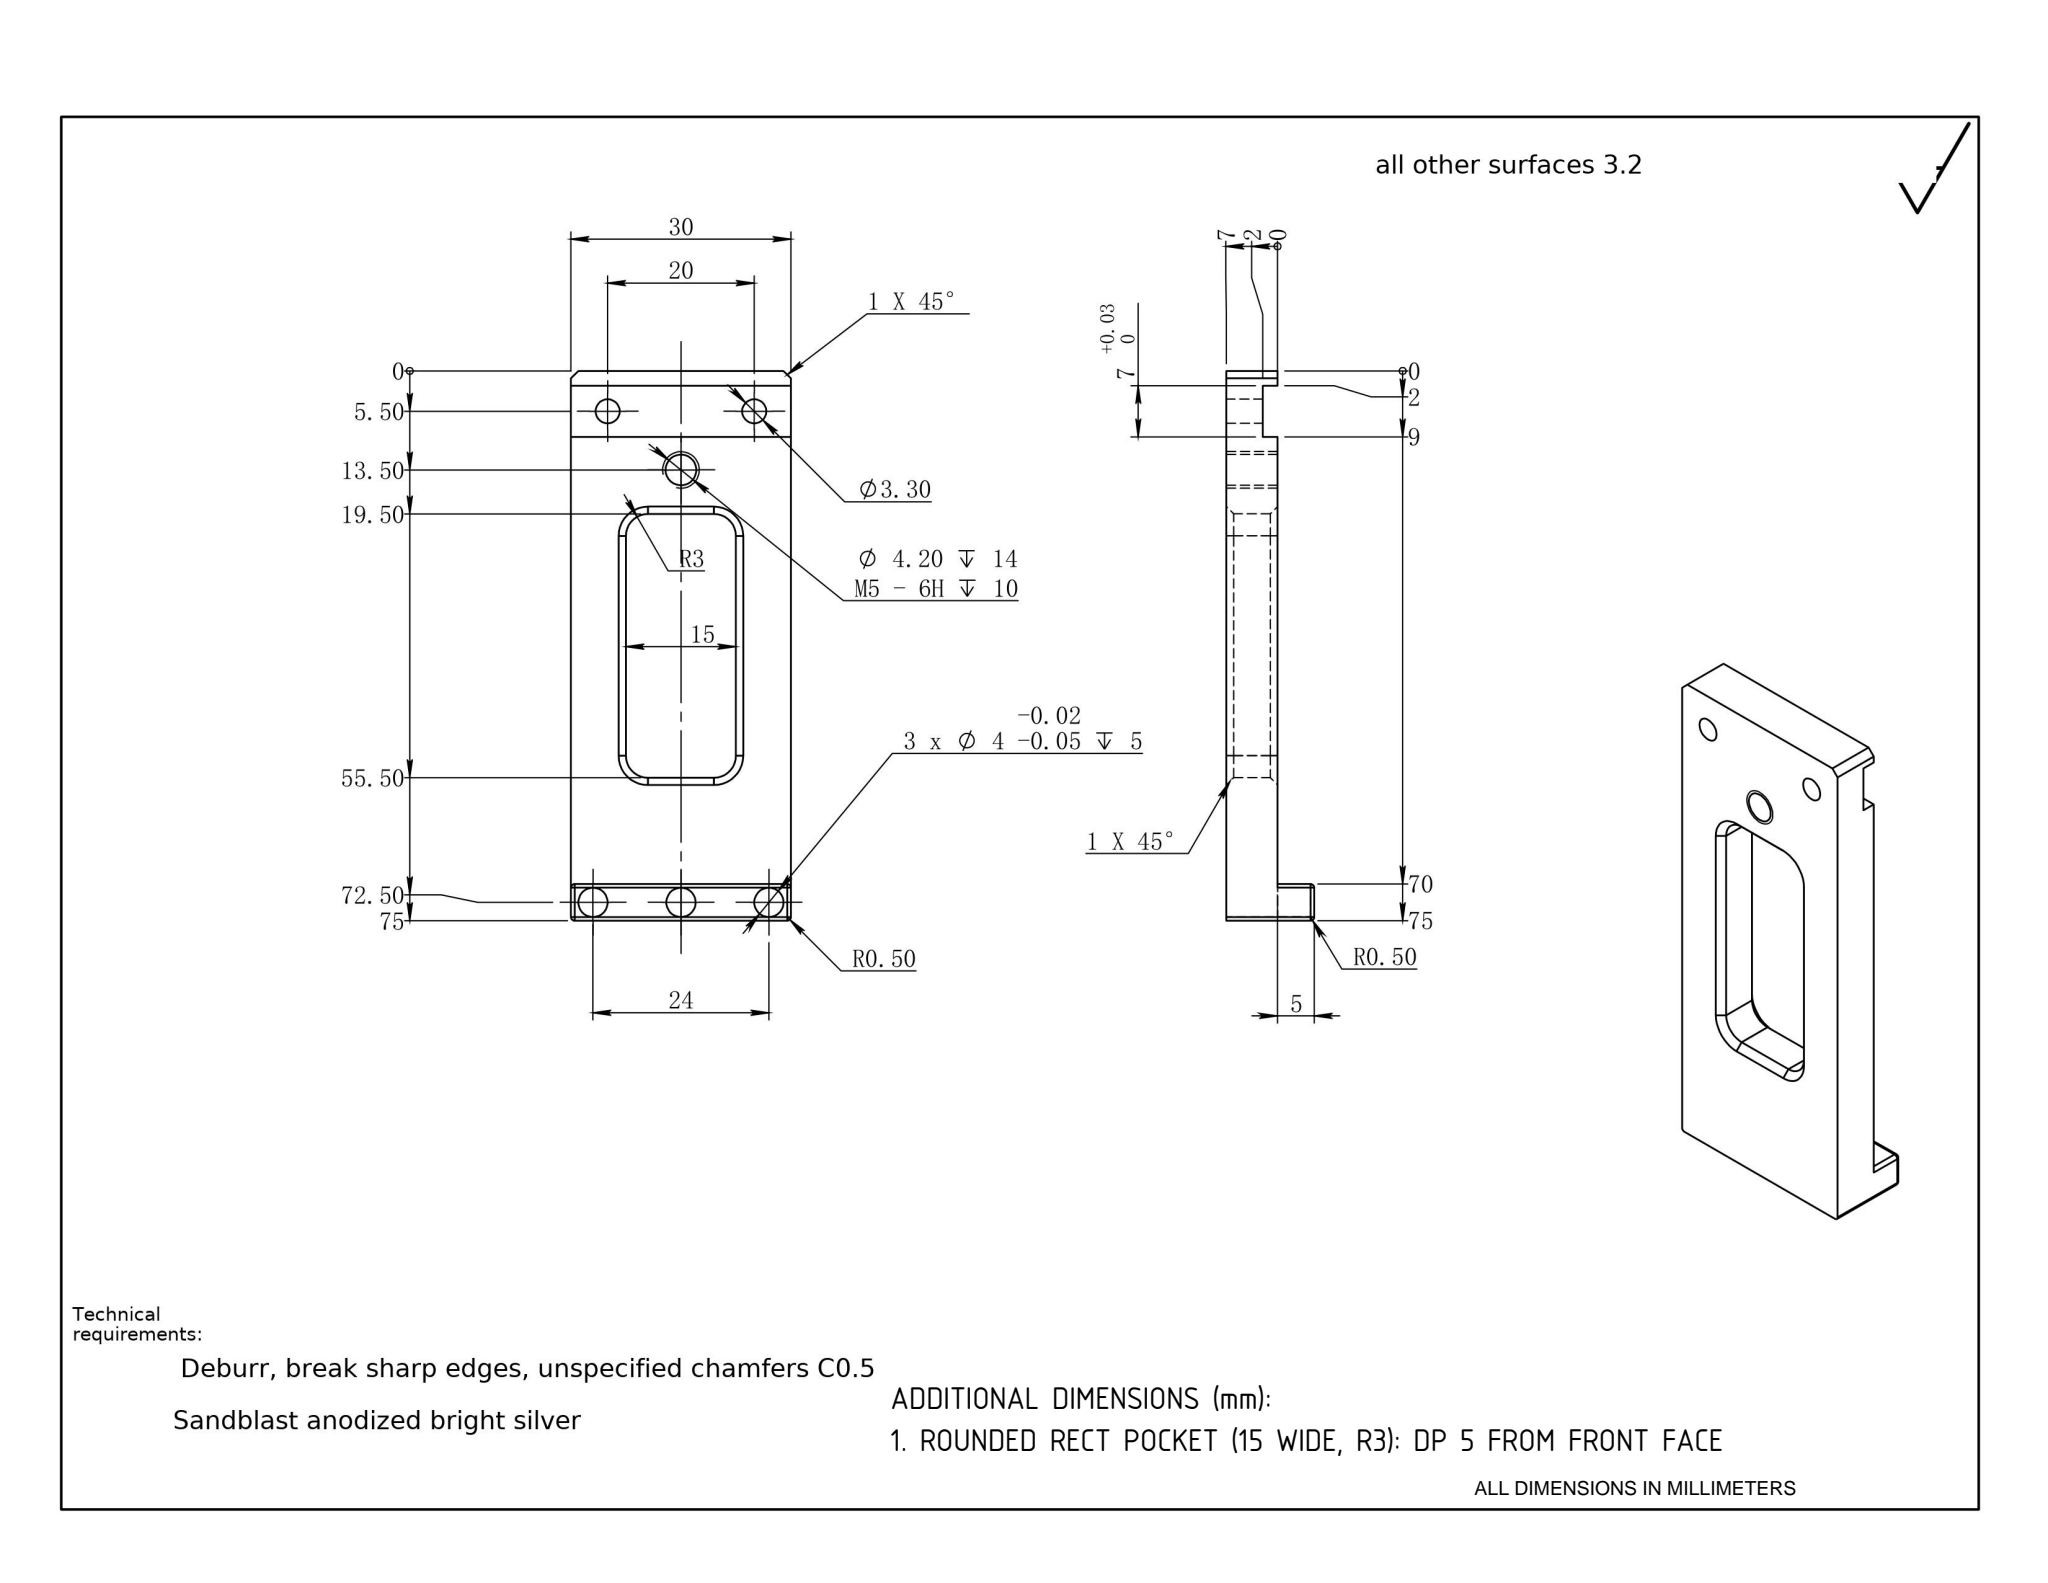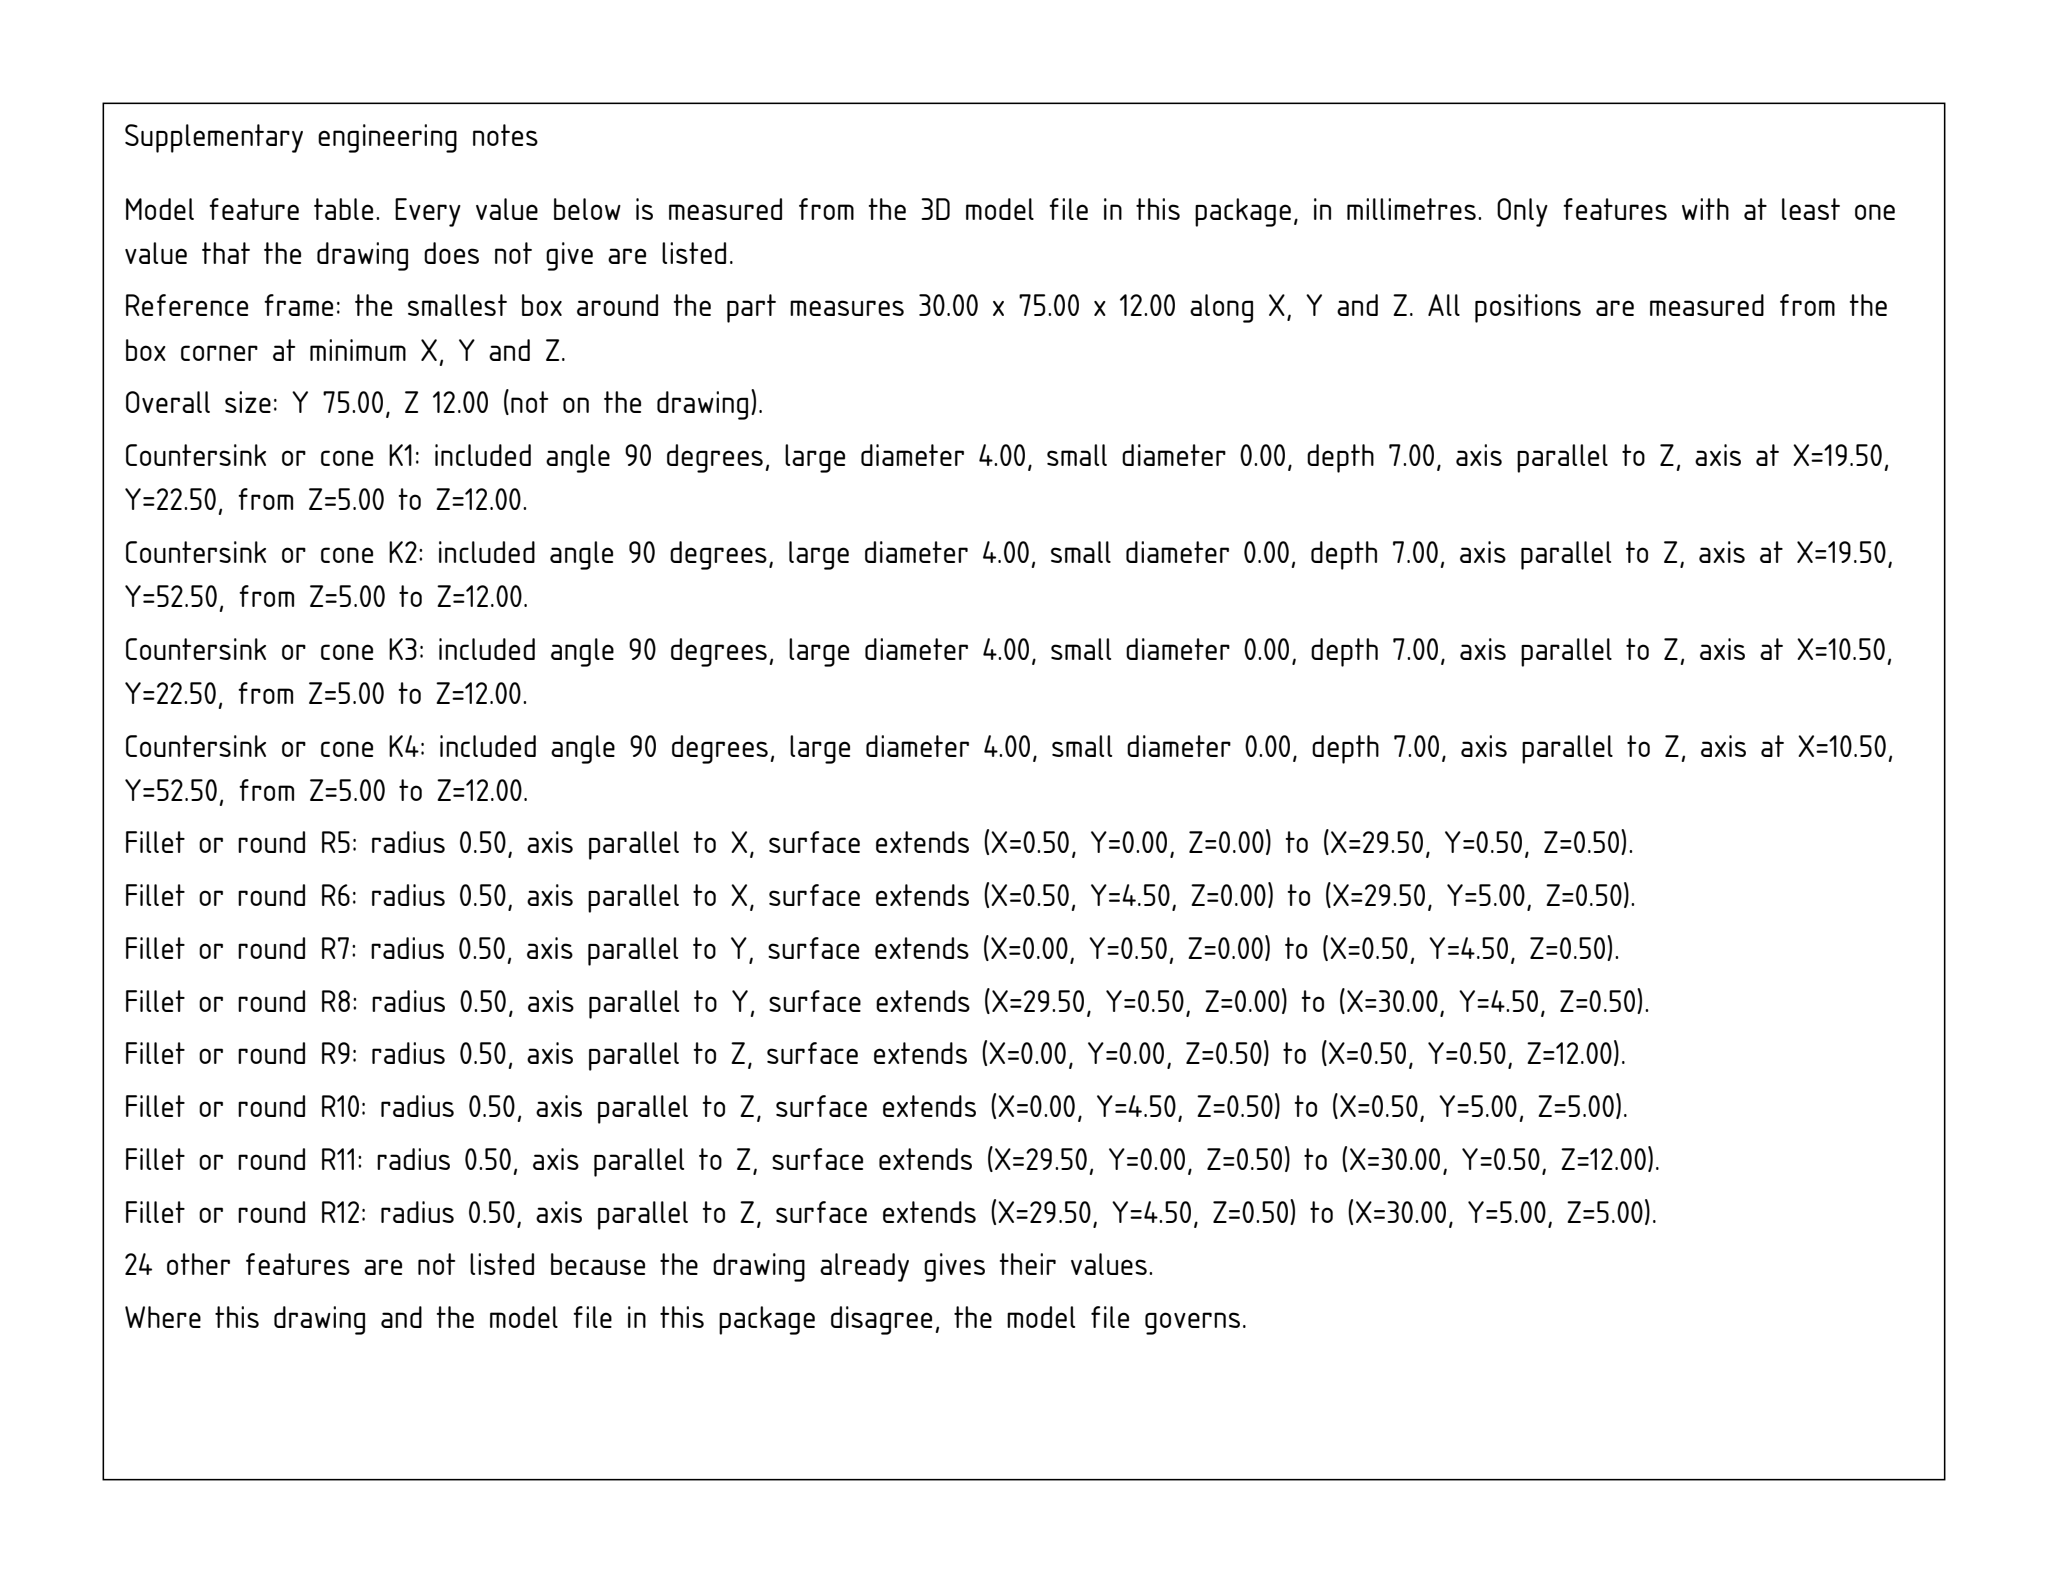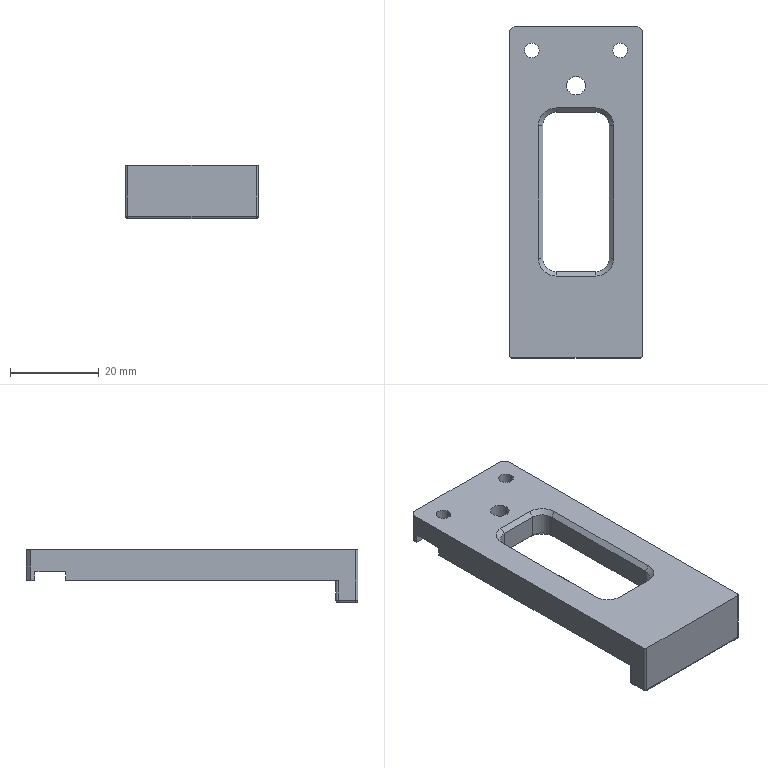Part | SolidWorks | mm | 1 solid | 68 faces | box 30 x 75 x 12 mm | volume 11872 mm3 | plane 32 | cylinder 24 | cone 8 | sphere 4 | commonest cylinder face diameters 1 x8 4 x6 3.3 x4 6 x4 4.2 x2
build123d program:
from build123d import *

# Parameters (mm, degrees)
SKETCH1_W                    = 30
SKETCH1_H                    = 75
BOSS_EXTRUDE1_DEPTH          = 3.5
SKETCH2_W                    = 30
SKETCH2_H                    = 5
BOSS_EXTRUDE2_DEPTH          = 5
SKETCH3_W                    = 30
SKETCH3_H                    = 7
CUT_EXTRUDE1_DEPTH           = 2
FILLET1_R                    = 0.5
F_3_3_3_3_DIAMETER_HOLE2_D   = 3.3
FILLET2_R                    = 0.5
F_4_0_4_DIAMETER_HOLE1_D     = 4
F_4_0_4_DIAMETER_HOLE1_DEPTH = 5
CHAMFER1_SIZE                = 1
SKETCH10_W                   = 15
SKETCH10_H                   = 36
CUT_EXTRUDE2_DEPTH           = 43.134
FILLET3_R                    = 3
CHAMFER2_SIZE                = 1
M5_TAPPED_HOLE1_D            = 4.2
M5_TAPPED_HOLE1_DEPTH        = 14
M5_TAPPED_HOLE1_TIP          = 1.262


with BuildPart() as part:
    # Sketch1 → Boss-Extrude1 (new, symmetric)
    with BuildSketch(Plane.XY):
        Rectangle(SKETCH1_W, SKETCH1_H)
    extrude(amount=BOSS_EXTRUDE1_DEPTH, both=True)

    # Sketch2 → Boss-Extrude2 (add)
    with BuildSketch(Plane(origin=(0, 0, -3.5), x_dir=(-1, 0, 0), z_dir=(0, 0, -1))):
        with Locations((0, -35)):
            Rectangle(SKETCH2_W, SKETCH2_H)
    extrude(amount=BOSS_EXTRUDE2_DEPTH)

    # Sketch3 → Cut-Extrude1 (cut)
    with BuildSketch(Plane(origin=(0, 0, -3.5), x_dir=(-1, 0, 0), z_dir=(0, 0, -1))):
        with Locations((0, 32)):
            Rectangle(SKETCH3_W, SKETCH3_H)
    extrude(amount=-CUT_EXTRUDE1_DEPTH, mode=Mode.SUBTRACT)

    # Fillet1
    fillet1_edges = [part.edges().sort_by_distance(p)[0] for p in [
        (0, -32.5, -8.5),
        (0, -37.5, -8.5),
    ]]
    fillet(fillet1_edges, radius=FILLET1_R)

    # 3.3 _3.3_ Diameter Hole2 (through all)
    with Locations(Plane.XY.offset(3.5)):
        with Locations((10, 32), (-10, 32)):
            Hole(F_3_3_3_3_DIAMETER_HOLE2_D / 2)

    # Fillet2
    fillet2_edges = [part.edges().sort_by_distance(p)[0] for p in [
        (-15, -37.5, -2.25),
        (-15, -37.354, -8.354),
        (-15, -35, -8.5),
        (-15, -32.646, -8.354),
        (15, -37.5, -2.25),
        (15, -37.354, -8.354),
        (15, -35, -8.5),
        (15, -32.646, -8.354),
        (-15, -32.5, -5.75),
        (15, -32.5, -5.75),
    ]]
    fillet(fillet2_edges, radius=FILLET2_R)

    # 4.0 _4_ Diameter Hole1
    with Locations(Plane(origin=(0, 0, -8.5), x_dir=(-1, 0, 0), z_dir=(0, 0, -1))):
        with Locations((-12, -35), (0, -35), (12, -35)):
            Hole(F_4_0_4_DIAMETER_HOLE1_D / 2, depth=F_4_0_4_DIAMETER_HOLE1_DEPTH)

    # Chamfer1
    chamfer1_edges = [part.edges().sort_by_distance(p)[0] for p in [
        (-15, 37.5, 0),
        (15, 37.5, 0),
    ]]
    chamfer(chamfer1_edges, length=CHAMFER1_SIZE)

    # Sketch10 → Cut-Extrude2 (cut, through all)
    with BuildSketch(Plane.XY.offset(3.5)):
        Rectangle(SKETCH10_W, SKETCH10_H)
    extrude(amount=-CUT_EXTRUDE2_DEPTH, mode=Mode.SUBTRACT)

    # Fillet3
    fillet3_edges = [part.edges().sort_by_distance(p)[0] for p in [
        (7.5, 18, 0),
        (7.5, -18, 0),
        (-7.5, -18, 0),
        (-7.5, 18, 0),
    ]]
    fillet(fillet3_edges, radius=FILLET3_R)

    # Chamfer2
    chamfer2_edges = [part.edges().sort_by_distance(p)[0] for p in [
        (0, -18, 3.5),
        (0, -18, -3.5),
        (-7.5, 0, 3.5),
        (-7.5, 0, -3.5),
        (7.5, 0, 3.5),
        (7.5, 0, -3.5),
        (0, 18, 3.5),
        (0, 18, -3.5),
        (-6.621, -17.121, 3.5),
        (-6.621, -17.121, -3.5),
        (6.621, -17.121, 3.5),
        (6.621, -17.121, -3.5),
        (6.621, 17.121, 3.5),
        (6.621, 17.121, -3.5),
        (-6.621, 17.121, 3.5),
        (-6.621, 17.121, -3.5),
    ]]
    chamfer(chamfer2_edges, length=CHAMFER2_SIZE)

    # M5 Tapped Hole1
    with Locations(Plane.XY.offset(3.5)):
        with Locations((0, 24)):
            Hole(M5_TAPPED_HOLE1_D / 2, depth=M5_TAPPED_HOLE1_DEPTH)
            with Locations((0, 0, -(M5_TAPPED_HOLE1_DEPTH + M5_TAPPED_HOLE1_TIP / 2))):  # 118° drill point
                Cone(0, M5_TAPPED_HOLE1_D / 2, M5_TAPPED_HOLE1_TIP, mode=Mode.SUBTRACT)


solid = part.part